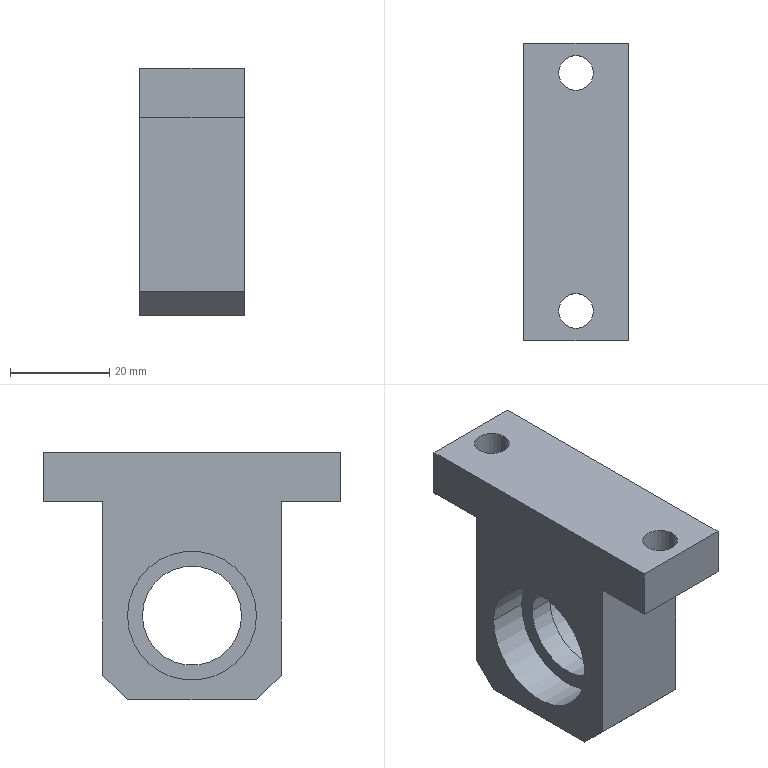Component | SolidWorks | VerticalFrontSeat-2-1 | 1 solid | 24 faces | box 21 x 60 x 50 mm | volume 31480 mm3 | plane 14 | cylinder 10 | commonest cylinder face diameters 7 x4 26 x4 20 x2
build123d program:
from build123d import *

# Parameters (mm, degrees)
SKETCH1_R           = 10
BOSS_EXTRUDE1_DEPTH = 21
SKETCH2_R           = 13
CUT_EXTRUDE1_DEPTH  = 8
CUT_EXTRUDE2_START  = -8
SKETCH3_R           = 13
CUT_EXTRUDE2_DEPTH  = 8
CHAMFER1_SIZE       = 5
SKETCH4_R           = 3.5
CUT_EXTRUDE3_DEPTH  = 12


with BuildPart() as part:
    # Sketch1 → Boss-Extrude1 (new body)
    with BuildSketch(Plane.XY):
        Polygon((12, 50), (12, 10), (0, 10), (0, 0), (60, 0), (60, 10), (48, 10), (48, 50), align=None)
        with Locations(Location((30, 33, 0), (0, 0, 180))):
            Circle(SKETCH1_R, mode=Mode.SUBTRACT)
    extrude(amount=BOSS_EXTRUDE1_DEPTH)

    # Sketch2 → Cut-Extrude1 (cut)
    with BuildSketch(Plane.XY.offset(21)):
        with Locations((30, 33)):
            Circle(SKETCH2_R)
    extrude(amount=-CUT_EXTRUDE1_DEPTH, mode=Mode.SUBTRACT)

    # Sketch3 → Cut-Extrude2 (cut)
    with BuildSketch(Plane(origin=(0, 0, 0), x_dir=(-1, 0, 0), z_dir=(0, 0, -1)).offset(CUT_EXTRUDE2_START)):
        with Locations(Location((-30, 33, 0), (0, 0, 180))):
            Circle(SKETCH3_R)
    extrude(amount=CUT_EXTRUDE2_DEPTH, mode=Mode.SUBTRACT)

    # Chamfer1
    chamfer1_edges = [part.edges().sort_by_distance(p)[0] for p in [
        (12, 50, 10.5),
        (48, 50, 10.5),
    ]]
    chamfer(chamfer1_edges, length=CHAMFER1_SIZE)

    # Sketch4 → Cut-Extrude3 (cut)
    with BuildSketch(Plane(origin=(0, 10, 0), x_dir=(1, 0, 0), z_dir=(0, 1, 0))):
        with Locations(Location((54, -10.5, 0), (0, 0, 270))):
            Circle(SKETCH4_R)
        with Locations(Location((6, -10.5, 0), (0, 0, 270))):
            Circle(SKETCH4_R)
    extrude(amount=-CUT_EXTRUDE3_DEPTH, mode=Mode.SUBTRACT)


solid = part.part

# Placed as in the assembly
solid = solid.moved(Location((28.978, 49.945, 36.551), (-90, 90, 0)))
STEP:
#1=COLOUR_RGB('',0.7922,0.8196,0.9333);
#2=FILL_AREA_STYLE_COLOUR('',#1);
#3=FILL_AREA_STYLE('',(#2));
#4=SURFACE_STYLE_FILL_AREA(#3);
#5=SURFACE_SIDE_STYLE('',(#4));
#6=SURFACE_STYLE_USAGE(.BOTH.,#5);
#7=PRESENTATION_STYLE_ASSIGNMENT((#6));
#8=CARTESIAN_POINT('',(1.692,-0.1596,1.439));
#9=VERTEX_POINT('',#8);
#10=CARTESIAN_POINT('',(1.416,-0.1596,1.439));
#11=VERTEX_POINT('',#10);
#12=CARTESIAN_POINT('',(1.554,-0.1596,1.439));
#13=DIRECTION('',(0.,0.,-1.));
#14=DIRECTION('',(-1.,0.,0.));
#15=AXIS2_PLACEMENT_3D('',#12,#13,#14);
#16=CIRCLE('',#15,0.1378);
#17=EDGE_CURVE('',#9,#11,#16,.T.);
#18=ORIENTED_EDGE('',*,*,#17,.F.);
#19=CARTESIAN_POINT('',(1.692,-0.1596,1.045));
#20=VERTEX_POINT('',#19);
#21=CARTESIAN_POINT('',(1.692,-0.1596,1.518));
#22=DIRECTION('',(0.,0.,-1.));
#23=VECTOR('',#22,39.37);
#24=LINE('',#21,#23);
#25=EDGE_CURVE('',#9,#20,#24,.T.);
#26=ORIENTED_EDGE('',*,*,#25,.T.);
#27=CARTESIAN_POINT('',(1.416,-0.1596,1.045));
#28=VERTEX_POINT('',#27);
#29=CARTESIAN_POINT('',(1.554,-0.1596,1.045));
#30=DIRECTION('',(0.,0.,-1.));
#31=DIRECTION('',(-1.,0.,0.));
#32=AXIS2_PLACEMENT_3D('',#29,#30,#31);
#33=CIRCLE('',#32,0.1378);
#34=EDGE_CURVE('',#20,#28,#33,.T.);
#35=ORIENTED_EDGE('',*,*,#34,.T.);
#36=CARTESIAN_POINT('',(1.416,-0.1596,1.518));
#37=DIRECTION('',(0.,0.,-1.));
#38=VECTOR('',#37,39.37);
#39=LINE('',#36,#38);
#40=EDGE_CURVE('',#11,#28,#39,.T.);
#41=ORIENTED_EDGE('',*,*,#40,.F.);
#42=EDGE_LOOP('',(#18,#26,#35,#41));
#43=FACE_OUTER_BOUND('',#42,.T.);
#44=CARTESIAN_POINT('',(1.554,-0.1596,1.518));
#45=DIRECTION('',(0.,0.,-1.));
#46=DIRECTION('',(-1.,0.,0.));
#47=AXIS2_PLACEMENT_3D('',#44,#45,#46);
#48=CYLINDRICAL_SURFACE('',#47,0.1378);
#49=ADVANCED_FACE('',(#43),#48,.F.);
#50=CARTESIAN_POINT('',(1.692,1.73,1.439));
#51=VERTEX_POINT('',#50);
#52=CARTESIAN_POINT('',(1.416,1.73,1.439));
#53=VERTEX_POINT('',#52);
#54=CARTESIAN_POINT('',(1.554,1.73,1.439));
#55=DIRECTION('',(0.,0.,-1.));
#56=DIRECTION('',(-1.,0.,0.));
#57=AXIS2_PLACEMENT_3D('',#54,#55,#56);
#58=CIRCLE('',#57,0.1378);
#59=EDGE_CURVE('',#51,#53,#58,.T.);
#60=ORIENTED_EDGE('',*,*,#59,.F.);
#61=CARTESIAN_POINT('',(1.692,1.73,1.045));
#62=VERTEX_POINT('',#61);
#63=CARTESIAN_POINT('',(1.692,1.73,1.518));
#64=DIRECTION('',(0.,0.,-1.));
#65=VECTOR('',#64,39.37);
#66=LINE('',#63,#65);
#67=EDGE_CURVE('',#51,#62,#66,.T.);
#68=ORIENTED_EDGE('',*,*,#67,.T.);
#69=CARTESIAN_POINT('',(1.416,1.73,1.045));
#70=VERTEX_POINT('',#69);
#71=CARTESIAN_POINT('',(1.554,1.73,1.045));
#72=DIRECTION('',(0.,0.,-1.));
#73=DIRECTION('',(-1.,0.,0.));
#74=AXIS2_PLACEMENT_3D('',#71,#72,#73);
#75=CIRCLE('',#74,0.1378);
#76=EDGE_CURVE('',#62,#70,#75,.T.);
#77=ORIENTED_EDGE('',*,*,#76,.T.);
#78=CARTESIAN_POINT('',(1.416,1.73,1.518));
#79=DIRECTION('',(0.,0.,-1.));
#80=VECTOR('',#79,39.37);
#81=LINE('',#78,#80);
#82=EDGE_CURVE('',#53,#70,#81,.T.);
#83=ORIENTED_EDGE('',*,*,#82,.F.);
#84=EDGE_LOOP('',(#60,#68,#77,#83));
#85=FACE_OUTER_BOUND('',#84,.T.);
#86=CARTESIAN_POINT('',(1.554,1.73,1.518));
#87=DIRECTION('',(0.,0.,-1.));
#88=DIRECTION('',(-1.,0.,0.));
#89=AXIS2_PLACEMENT_3D('',#86,#87,#88);
#90=CYLINDRICAL_SURFACE('',#89,0.1378);
#91=ADVANCED_FACE('',(#85),#90,.F.);
#92=CARTESIAN_POINT('',(1.653,1.297,0.1398));
#93=VERTEX_POINT('',#92);
#94=CARTESIAN_POINT('',(1.653,0.2734,0.1398));
#95=VERTEX_POINT('',#94);
#96=CARTESIAN_POINT('',(1.653,0.7853,0.1398));
#97=DIRECTION('',(1.,-0.,0.));
#98=DIRECTION('',(0.,-1.,-0.));
#99=AXIS2_PLACEMENT_3D('',#96,#97,#98);
#100=CIRCLE('',#99,0.5118);
#101=EDGE_CURVE('',#93,#95,#100,.T.);
#102=ORIENTED_EDGE('',*,*,#101,.F.);
#103=CARTESIAN_POINT('',(1.968,1.297,0.1398));
#104=VERTEX_POINT('',#103);
#105=CARTESIAN_POINT('',(1.653,1.297,0.1398));
#106=DIRECTION('',(1.,-0.,0.));
#107=VECTOR('',#106,39.37);
#108=LINE('',#105,#107);
#109=EDGE_CURVE('',#93,#104,#108,.T.);
#110=ORIENTED_EDGE('',*,*,#109,.T.);
#111=CARTESIAN_POINT('',(1.968,0.2734,0.1398));
#112=VERTEX_POINT('',#111);
#113=CARTESIAN_POINT('',(1.968,0.7853,0.1398));
#114=DIRECTION('',(1.,-0.,0.));
#115=DIRECTION('',(0.,-1.,-0.));
#116=AXIS2_PLACEMENT_3D('',#113,#114,#115);
#117=CIRCLE('',#116,0.5118);
#118=EDGE_CURVE('',#104,#112,#117,.T.);
#119=ORIENTED_EDGE('',*,*,#118,.T.);
#120=CARTESIAN_POINT('',(1.653,0.2734,0.1398));
#121=DIRECTION('',(1.,-0.,0.));
#122=VECTOR('',#121,39.37);
#123=LINE('',#120,#122);
#124=EDGE_CURVE('',#95,#112,#123,.T.);
#125=ORIENTED_EDGE('',*,*,#124,.F.);
#126=EDGE_LOOP('',(#102,#110,#119,#125));
#127=FACE_OUTER_BOUND('',#126,.T.);
#128=CARTESIAN_POINT('',(1.653,0.7853,0.1398));
#129=DIRECTION('',(1.,-0.,0.));
#130=DIRECTION('',(0.,-1.,-0.));
#131=AXIS2_PLACEMENT_3D('',#128,#129,#130);
#132=CYLINDRICAL_SURFACE('',#131,0.5118);
#133=ADVANCED_FACE('',(#127),#132,.F.);
#134=CARTESIAN_POINT('',(1.456,0.2734,0.1398));
#135=VERTEX_POINT('',#134);
#136=CARTESIAN_POINT('',(1.456,1.297,0.1398));
#137=VERTEX_POINT('',#136);
#138=CARTESIAN_POINT('',(1.456,0.7853,0.1398));
#139=DIRECTION('',(-1.,0.,-0.));
#140=DIRECTION('',(0.,1.,0.));
#141=AXIS2_PLACEMENT_3D('',#138,#139,#140);
#142=CIRCLE('',#141,0.5118);
#143=EDGE_CURVE('',#135,#137,#142,.T.);
#144=ORIENTED_EDGE('',*,*,#143,.F.);
#145=CARTESIAN_POINT('',(1.141,0.2734,0.1398));
#146=VERTEX_POINT('',#145);
#147=CARTESIAN_POINT('',(1.456,0.2734,0.1398));
#148=DIRECTION('',(-1.,0.,-0.));
#149=VECTOR('',#148,39.37);
#150=LINE('',#147,#149);
#151=EDGE_CURVE('',#135,#146,#150,.T.);
#152=ORIENTED_EDGE('',*,*,#151,.T.);
#153=CARTESIAN_POINT('',(1.141,1.297,0.1398));
#154=VERTEX_POINT('',#153);
#155=CARTESIAN_POINT('',(1.141,0.7853,0.1398));
#156=DIRECTION('',(-1.,0.,-0.));
#157=DIRECTION('',(0.,1.,0.));
#158=AXIS2_PLACEMENT_3D('',#155,#156,#157);
#159=CIRCLE('',#158,0.5118);
#160=EDGE_CURVE('',#146,#154,#159,.T.);
#161=ORIENTED_EDGE('',*,*,#160,.T.);
#162=CARTESIAN_POINT('',(1.456,1.297,0.1398));
#163=DIRECTION('',(-1.,0.,-0.));
#164=VECTOR('',#163,39.37);
#165=LINE('',#162,#164);
#166=EDGE_CURVE('',#137,#154,#165,.T.);
#167=ORIENTED_EDGE('',*,*,#166,.F.);
#168=EDGE_LOOP('',(#144,#152,#161,#167));
#169=FACE_OUTER_BOUND('',#168,.T.);
#170=CARTESIAN_POINT('',(1.456,0.7853,0.1398));
#171=DIRECTION('',(-1.,0.,-0.));
#172=DIRECTION('',(0.,1.,0.));
#173=AXIS2_PLACEMENT_3D('',#170,#171,#172);
#174=CYLINDRICAL_SURFACE('',#173,0.5118);
#175=ADVANCED_FACE('',(#169),#174,.F.);
#176=CARTESIAN_POINT('',(1.456,0.3916,0.1398));
#177=VERTEX_POINT('',#176);
#178=CARTESIAN_POINT('',(1.456,1.179,0.1398));
#179=VERTEX_POINT('',#178);
#180=CARTESIAN_POINT('',(1.456,0.7853,0.1398));
#181=DIRECTION('',(-1.,0.,-0.));
#182=DIRECTION('',(0.,1.,0.));
#183=AXIS2_PLACEMENT_3D('',#180,#181,#182);
#184=CIRCLE('',#183,0.3937);
#185=EDGE_CURVE('',#177,#179,#184,.T.);
#186=ORIENTED_EDGE('',*,*,#185,.T.);
#187=CARTESIAN_POINT('',(1.653,1.179,0.1398));
#188=VERTEX_POINT('',#187);
#189=CARTESIAN_POINT('',(1.141,1.179,0.1398));
#190=DIRECTION('',(1.,-0.,0.));
#191=VECTOR('',#190,39.37);
#192=LINE('',#189,#191);
#193=EDGE_CURVE('',#179,#188,#192,.T.);
#194=ORIENTED_EDGE('',*,*,#193,.T.);
#195=CARTESIAN_POINT('',(1.653,0.3916,0.1398));
#196=VERTEX_POINT('',#195);
#197=CARTESIAN_POINT('',(1.653,0.7853,0.1398));
#198=DIRECTION('',(1.,-0.,0.));
#199=DIRECTION('',(0.,-1.,0.));
#200=AXIS2_PLACEMENT_3D('',#197,#198,#199);
#201=CIRCLE('',#200,0.3937);
#202=EDGE_CURVE('',#188,#196,#201,.T.);
#203=ORIENTED_EDGE('',*,*,#202,.T.);
#204=CARTESIAN_POINT('',(1.141,0.3916,0.1398));
#205=DIRECTION('',(1.,-0.,0.));
#206=VECTOR('',#205,39.37);
#207=LINE('',#204,#206);
#208=EDGE_CURVE('',#177,#196,#207,.T.);
#209=ORIENTED_EDGE('',*,*,#208,.F.);
#210=EDGE_LOOP('',(#186,#194,#203,#209));
#211=FACE_OUTER_BOUND('',#210,.T.);
#212=CARTESIAN_POINT('',(1.141,0.7853,0.1398));
#213=DIRECTION('',(1.,-0.,0.));
#214=DIRECTION('',(0.,-1.,0.));
#215=AXIS2_PLACEMENT_3D('',#212,#213,#214);
#216=CYLINDRICAL_SURFACE('',#215,0.3937);
#217=ADVANCED_FACE('',(#211),#216,.F.);
#218=ORIENTED_EDGE('',*,*,#193,.F.);
#219=CARTESIAN_POINT('',(1.456,0.7853,0.1398));
#220=DIRECTION('',(-1.,0.,-0.));
#221=DIRECTION('',(0.,1.,0.));
#222=AXIS2_PLACEMENT_3D('',#219,#220,#221);
#223=CIRCLE('',#222,0.3937);
#224=EDGE_CURVE('',#179,#177,#223,.T.);
#225=ORIENTED_EDGE('',*,*,#224,.T.);
#226=ORIENTED_EDGE('',*,*,#208,.T.);
#227=CARTESIAN_POINT('',(1.653,0.7853,0.1398));
#228=DIRECTION('',(1.,-0.,0.));
#229=DIRECTION('',(0.,-1.,0.));
#230=AXIS2_PLACEMENT_3D('',#227,#228,#229);
#231=CIRCLE('',#230,0.3937);
#232=EDGE_CURVE('',#196,#188,#231,.T.);
#233=ORIENTED_EDGE('',*,*,#232,.T.);
#234=EDGE_LOOP('',(#218,#225,#226,#233));
#235=FACE_OUTER_BOUND('',#234,.T.);
#236=CARTESIAN_POINT('',(1.141,0.7853,0.1398));
#237=DIRECTION('',(1.,-0.,0.));
#238=DIRECTION('',(0.,-1.,0.));
#239=AXIS2_PLACEMENT_3D('',#236,#237,#238);
#240=CYLINDRICAL_SURFACE('',#239,0.3937);
#241=ADVANCED_FACE('',(#235),#240,.F.);
#242=CARTESIAN_POINT('',(1.141,0.7853,0.1398));
#243=DIRECTION('',(-1.,0.,-0.));
#244=DIRECTION('',(0.,1.,0.));
#245=AXIS2_PLACEMENT_3D('',#242,#243,#244);
#246=CIRCLE('',#245,0.5118);
#247=EDGE_CURVE('',#154,#146,#246,.T.);
#248=ORIENTED_EDGE('',*,*,#247,.F.);
#249=ORIENTED_EDGE('',*,*,#160,.F.);
#250=EDGE_LOOP('',(#248,#249));
#251=FACE_BOUND('',#250,.T.);
#252=CARTESIAN_POINT('',(1.141,1.297,-0.5295));
#253=VERTEX_POINT('',#252);
#254=CARTESIAN_POINT('',(1.141,0.2734,-0.5295));
#255=VERTEX_POINT('',#254);
#256=CARTESIAN_POINT('',(1.141,0.07659,-0.5295));
#257=DIRECTION('',(-0.,-1.,-0.));
#258=VECTOR('',#257,39.37);
#259=LINE('',#256,#258);
#260=EDGE_CURVE('',#253,#255,#259,.T.);
#261=ORIENTED_EDGE('',*,*,#260,.T.);
#262=CARTESIAN_POINT('',(1.141,0.07659,-0.3326));
#263=VERTEX_POINT('',#262);
#264=CARTESIAN_POINT('',(1.141,-1.045,0.7894));
#265=DIRECTION('',(-0.,-0.7071,0.7071));
#266=VECTOR('',#265,39.37);
#267=LINE('',#264,#266);
#268=EDGE_CURVE('',#255,#263,#267,.T.);
#269=ORIENTED_EDGE('',*,*,#268,.T.);
#270=CARTESIAN_POINT('',(1.141,0.07659,1.045));
#271=VERTEX_POINT('',#270);
#272=CARTESIAN_POINT('',(1.141,0.07659,-0.5295));
#273=DIRECTION('',(-0.,0.,1.));
#274=VECTOR('',#273,39.37);
#275=LINE('',#272,#274);
#276=EDGE_CURVE('',#263,#271,#275,.T.);
#277=ORIENTED_EDGE('',*,*,#276,.T.);
#278=CARTESIAN_POINT('',(1.141,-0.3959,1.045));
#279=VERTEX_POINT('',#278);
#280=CARTESIAN_POINT('',(1.141,0.07659,1.045));
#281=DIRECTION('',(-0.,-1.,0.));
#282=VECTOR('',#281,39.37);
#283=LINE('',#280,#282);
#284=EDGE_CURVE('',#271,#279,#283,.T.);
#285=ORIENTED_EDGE('',*,*,#284,.T.);
#286=CARTESIAN_POINT('',(1.141,-0.3959,1.439));
#287=VERTEX_POINT('',#286);
#288=CARTESIAN_POINT('',(1.141,-0.3959,1.439));
#289=DIRECTION('',(-0.,-0.,1.));
#290=VECTOR('',#289,39.37);
#291=LINE('',#288,#290);
#292=EDGE_CURVE('',#279,#287,#291,.T.);
#293=ORIENTED_EDGE('',*,*,#292,.T.);
#294=CARTESIAN_POINT('',(1.141,1.966,1.439));
#295=VERTEX_POINT('',#294);
#296=CARTESIAN_POINT('',(1.141,-0.3959,1.439));
#297=DIRECTION('',(0.,1.,0.));
#298=VECTOR('',#297,39.37);
#299=LINE('',#296,#298);
#300=EDGE_CURVE('',#287,#295,#299,.T.);
#301=ORIENTED_EDGE('',*,*,#300,.T.);
#302=CARTESIAN_POINT('',(1.141,1.966,1.045));
#303=VERTEX_POINT('',#302);
#304=CARTESIAN_POINT('',(1.141,1.966,1.439));
#305=DIRECTION('',(0.,0.,-1.));
#306=VECTOR('',#305,39.37);
#307=LINE('',#304,#306);
#308=EDGE_CURVE('',#295,#303,#307,.T.);
#309=ORIENTED_EDGE('',*,*,#308,.T.);
#310=CARTESIAN_POINT('',(1.141,1.494,1.045));
#311=VERTEX_POINT('',#310);
#312=CARTESIAN_POINT('',(1.141,1.494,1.045));
#313=DIRECTION('',(-0.,-1.,-0.));
#314=VECTOR('',#313,39.37);
#315=LINE('',#312,#314);
#316=EDGE_CURVE('',#303,#311,#315,.T.);
#317=ORIENTED_EDGE('',*,*,#316,.T.);
#318=CARTESIAN_POINT('',(1.141,1.494,-0.3326));
#319=VERTEX_POINT('',#318);
#320=CARTESIAN_POINT('',(1.141,1.494,-0.5295));
#321=DIRECTION('',(0.,-0.,-1.));
#322=VECTOR('',#321,39.37);
#323=LINE('',#320,#322);
#324=EDGE_CURVE('',#311,#319,#323,.T.);
#325=ORIENTED_EDGE('',*,*,#324,.T.);
#326=CARTESIAN_POINT('',(1.141,1.435,-0.3917));
#327=DIRECTION('',(-0.,-0.7071,-0.7071));
#328=VECTOR('',#327,39.37);
#329=LINE('',#326,#328);
#330=EDGE_CURVE('',#319,#253,#329,.T.);
#331=ORIENTED_EDGE('',*,*,#330,.T.);
#332=EDGE_LOOP('',(#261,#269,#277,#285,#293,#301,#309,#317,#325,#331));
#333=FACE_OUTER_BOUND('',#332,.T.);
#334=CARTESIAN_POINT('',(1.141,-0.3959,1.439));
#335=DIRECTION('',(-1.,0.,-0.));
#336=DIRECTION('',(0.,1.,0.));
#337=AXIS2_PLACEMENT_3D('',#334,#335,#336);
#338=PLANE('',#337);
#339=ADVANCED_FACE('',(#251,#333),#338,.T.);
#340=CARTESIAN_POINT('',(1.968,0.7853,0.1398));
#341=DIRECTION('',(1.,-0.,0.));
#342=DIRECTION('',(0.,-1.,-0.));
#343=AXIS2_PLACEMENT_3D('',#340,#341,#342);
#344=CIRCLE('',#343,0.5118);
#345=EDGE_CURVE('',#112,#104,#344,.T.);
#346=ORIENTED_EDGE('',*,*,#345,.F.);
#347=ORIENTED_EDGE('',*,*,#118,.F.);
#348=EDGE_LOOP('',(#346,#347));
#349=FACE_BOUND('',#348,.T.);
#350=CARTESIAN_POINT('',(1.968,0.07659,-0.3326));
#351=VERTEX_POINT('',#350);
#352=CARTESIAN_POINT('',(1.968,0.07659,1.045));
#353=VERTEX_POINT('',#352);
#354=CARTESIAN_POINT('',(1.968,0.07659,-0.5295));
#355=DIRECTION('',(-0.,0.,1.));
#356=VECTOR('',#355,39.37);
#357=LINE('',#354,#356);
#358=EDGE_CURVE('',#351,#353,#357,.T.);
#359=ORIENTED_EDGE('',*,*,#358,.F.);
#360=CARTESIAN_POINT('',(1.968,0.2734,-0.5295));
#361=VERTEX_POINT('',#360);
#362=CARTESIAN_POINT('',(1.968,0.07659,-0.3326));
#363=DIRECTION('',(0.,0.7071,-0.7071));
#364=VECTOR('',#363,39.37);
#365=LINE('',#362,#364);
#366=EDGE_CURVE('',#351,#361,#365,.T.);
#367=ORIENTED_EDGE('',*,*,#366,.T.);
#368=CARTESIAN_POINT('',(1.968,1.297,-0.5295));
#369=VERTEX_POINT('',#368);
#370=CARTESIAN_POINT('',(1.968,0.07659,-0.5295));
#371=DIRECTION('',(-0.,-1.,-0.));
#372=VECTOR('',#371,39.37);
#373=LINE('',#370,#372);
#374=EDGE_CURVE('',#369,#361,#373,.T.);
#375=ORIENTED_EDGE('',*,*,#374,.F.);
#376=CARTESIAN_POINT('',(1.968,1.494,-0.3326));
#377=VERTEX_POINT('',#376);
#378=CARTESIAN_POINT('',(1.968,1.297,-0.5295));
#379=DIRECTION('',(0.,0.7071,0.7071));
#380=VECTOR('',#379,39.37);
#381=LINE('',#378,#380);
#382=EDGE_CURVE('',#369,#377,#381,.T.);
#383=ORIENTED_EDGE('',*,*,#382,.T.);
#384=CARTESIAN_POINT('',(1.968,1.494,1.045));
#385=VERTEX_POINT('',#384);
#386=CARTESIAN_POINT('',(1.968,1.494,-0.5295));
#387=DIRECTION('',(0.,-0.,-1.));
#388=VECTOR('',#387,39.37);
#389=LINE('',#386,#388);
#390=EDGE_CURVE('',#385,#377,#389,.T.);
#391=ORIENTED_EDGE('',*,*,#390,.F.);
#392=CARTESIAN_POINT('',(1.968,1.966,1.045));
#393=VERTEX_POINT('',#392);
#394=CARTESIAN_POINT('',(1.968,1.494,1.045));
#395=DIRECTION('',(-0.,-1.,-0.));
#396=VECTOR('',#395,39.37);
#397=LINE('',#394,#396);
#398=EDGE_CURVE('',#393,#385,#397,.T.);
#399=ORIENTED_EDGE('',*,*,#398,.F.);
#400=CARTESIAN_POINT('',(1.968,1.966,1.439));
#401=VERTEX_POINT('',#400);
#402=CARTESIAN_POINT('',(1.968,1.966,1.439));
#403=DIRECTION('',(0.,0.,-1.));
#404=VECTOR('',#403,39.37);
#405=LINE('',#402,#404);
#406=EDGE_CURVE('',#401,#393,#405,.T.);
#407=ORIENTED_EDGE('',*,*,#406,.F.);
#408=CARTESIAN_POINT('',(1.968,-0.3959,1.439));
#409=VERTEX_POINT('',#408);
#410=CARTESIAN_POINT('',(1.968,-0.3959,1.439));
#411=DIRECTION('',(0.,1.,0.));
#412=VECTOR('',#411,39.37);
#413=LINE('',#410,#412);
#414=EDGE_CURVE('',#409,#401,#413,.T.);
#415=ORIENTED_EDGE('',*,*,#414,.F.);
#416=CARTESIAN_POINT('',(1.968,-0.3959,1.045));
#417=VERTEX_POINT('',#416);
#418=CARTESIAN_POINT('',(1.968,-0.3959,1.439));
#419=DIRECTION('',(-0.,-0.,1.));
#420=VECTOR('',#419,39.37);
#421=LINE('',#418,#420);
#422=EDGE_CURVE('',#417,#409,#421,.T.);
#423=ORIENTED_EDGE('',*,*,#422,.F.);
#424=CARTESIAN_POINT('',(1.968,0.07659,1.045));
#425=DIRECTION('',(-0.,-1.,0.));
#426=VECTOR('',#425,39.37);
#427=LINE('',#424,#426);
#428=EDGE_CURVE('',#353,#417,#427,.T.);
#429=ORIENTED_EDGE('',*,*,#428,.F.);
#430=EDGE_LOOP('',(#359,#367,#375,#383,#391,#399,#407,#415,#423,#429));
#431=FACE_OUTER_BOUND('',#430,.T.);
#432=CARTESIAN_POINT('',(1.968,-0.3959,1.439));
#433=DIRECTION('',(-1.,0.,-0.));
#434=DIRECTION('',(0.,1.,0.));
#435=AXIS2_PLACEMENT_3D('',#432,#433,#434);
#436=PLANE('',#435);
#437=ADVANCED_FACE('',(#349,#431),#436,.F.);
#438=ORIENTED_EDGE('',*,*,#422,.T.);
#439=CARTESIAN_POINT('',(1.141,-0.3959,1.439));
#440=DIRECTION('',(1.,-0.,0.));
#441=VECTOR('',#440,39.37);
#442=LINE('',#439,#441);
#443=EDGE_CURVE('',#287,#409,#442,.T.);
#444=ORIENTED_EDGE('',*,*,#443,.F.);
#445=ORIENTED_EDGE('',*,*,#292,.F.);
#446=CARTESIAN_POINT('',(1.141,-0.3959,1.045));
#447=DIRECTION('',(1.,-0.,0.));
#448=VECTOR('',#447,39.37);
#449=LINE('',#446,#448);
#450=EDGE_CURVE('',#279,#417,#449,.T.);
#451=ORIENTED_EDGE('',*,*,#450,.T.);
#452=EDGE_LOOP('',(#438,#444,#445,#451));
#453=FACE_OUTER_BOUND('',#452,.T.);
#454=CARTESIAN_POINT('',(1.141,-0.3959,1.439));
#455=DIRECTION('',(0.,1.,0.));
#456=DIRECTION('',(1.,-0.,0.));
#457=AXIS2_PLACEMENT_3D('',#454,#455,#456);
#458=PLANE('',#457);
#459=ADVANCED_FACE('',(#453),#458,.F.);
#460=CARTESIAN_POINT('',(1.554,-0.1596,1.439));
#461=DIRECTION('',(0.,0.,-1.));
#462=DIRECTION('',(-1.,0.,0.));
#463=AXIS2_PLACEMENT_3D('',#460,#461,#462);
#464=CIRCLE('',#463,0.1378);
#465=EDGE_CURVE('',#11,#9,#464,.T.);
#466=ORIENTED_EDGE('',*,*,#465,.T.);
#467=ORIENTED_EDGE('',*,*,#17,.T.);
#468=EDGE_LOOP('',(#466,#467));
#469=FACE_BOUND('',#468,.T.);
#470=CARTESIAN_POINT('',(1.554,1.73,1.439));
#471=DIRECTION('',(0.,0.,-1.));
#472=DIRECTION('',(-1.,0.,0.));
#473=AXIS2_PLACEMENT_3D('',#470,#471,#472);
#474=CIRCLE('',#473,0.1378);
#475=EDGE_CURVE('',#53,#51,#474,.T.);
#476=ORIENTED_EDGE('',*,*,#475,.T.);
#477=ORIENTED_EDGE('',*,*,#59,.T.);
#478=EDGE_LOOP('',(#476,#477));
#479=FACE_BOUND('',#478,.T.);
#480=ORIENTED_EDGE('',*,*,#414,.T.);
#481=CARTESIAN_POINT('',(1.141,1.966,1.439));
#482=DIRECTION('',(1.,-0.,0.));
#483=VECTOR('',#482,39.37);
#484=LINE('',#481,#483);
#485=EDGE_CURVE('',#295,#401,#484,.T.);
#486=ORIENTED_EDGE('',*,*,#485,.F.);
#487=ORIENTED_EDGE('',*,*,#300,.F.);
#488=ORIENTED_EDGE('',*,*,#443,.T.);
#489=EDGE_LOOP('',(#480,#486,#487,#488));
#490=FACE_OUTER_BOUND('',#489,.T.);
#491=CARTESIAN_POINT('',(1.141,-0.3959,1.439));
#492=DIRECTION('',(0.,0.,-1.));
#493=DIRECTION('',(-1.,0.,-0.));
#494=AXIS2_PLACEMENT_3D('',#491,#492,#493);
#495=PLANE('',#494);
#496=ADVANCED_FACE('',(#469,#479,#490),#495,.F.);
#497=ORIENTED_EDGE('',*,*,#406,.T.);
#498=CARTESIAN_POINT('',(1.141,1.966,1.045));
#499=DIRECTION('',(1.,-0.,0.));
#500=VECTOR('',#499,39.37);
#501=LINE('',#498,#500);
#502=EDGE_CURVE('',#303,#393,#501,.T.);
#503=ORIENTED_EDGE('',*,*,#502,.F.);
#504=ORIENTED_EDGE('',*,*,#308,.F.);
#505=ORIENTED_EDGE('',*,*,#485,.T.);
#506=EDGE_LOOP('',(#497,#503,#504,#505));
#507=FACE_OUTER_BOUND('',#506,.T.);
#508=CARTESIAN_POINT('',(1.141,1.966,1.439));
#509=DIRECTION('',(-0.,-1.,-0.));
#510=DIRECTION('',(-1.,0.,-0.));
#511=AXIS2_PLACEMENT_3D('',#508,#509,#510);
#512=PLANE('',#511);
#513=ADVANCED_FACE('',(#507),#512,.F.);
#514=CARTESIAN_POINT('',(1.554,1.73,1.045));
#515=DIRECTION('',(0.,0.,-1.));
#516=DIRECTION('',(-1.,0.,0.));
#517=AXIS2_PLACEMENT_3D('',#514,#515,#516);
#518=CIRCLE('',#517,0.1378);
#519=EDGE_CURVE('',#70,#62,#518,.T.);
#520=ORIENTED_EDGE('',*,*,#519,.F.);
#521=ORIENTED_EDGE('',*,*,#76,.F.);
#522=EDGE_LOOP('',(#520,#521));
#523=FACE_BOUND('',#522,.T.);
#524=ORIENTED_EDGE('',*,*,#398,.T.);
#525=CARTESIAN_POINT('',(1.141,1.494,1.045));
#526=DIRECTION('',(1.,-0.,0.));
#527=VECTOR('',#526,39.37);
#528=LINE('',#525,#527);
#529=EDGE_CURVE('',#311,#385,#528,.T.);
#530=ORIENTED_EDGE('',*,*,#529,.F.);
#531=ORIENTED_EDGE('',*,*,#316,.F.);
#532=ORIENTED_EDGE('',*,*,#502,.T.);
#533=EDGE_LOOP('',(#524,#530,#531,#532));
#534=FACE_OUTER_BOUND('',#533,.T.);
#535=CARTESIAN_POINT('',(1.141,1.494,1.045));
#536=DIRECTION('',(-0.,-0.,1.));
#537=DIRECTION('',(1.,-0.,0.));
#538=AXIS2_PLACEMENT_3D('',#535,#536,#537);
#539=PLANE('',#538);
#540=ADVANCED_FACE('',(#523,#534),#539,.F.);
#541=ORIENTED_EDGE('',*,*,#390,.T.);
#542=CARTESIAN_POINT('',(1.141,1.494,-0.3326));
#543=DIRECTION('',(-1.,0.,-0.));
#544=VECTOR('',#543,39.37);
#545=LINE('',#542,#544);
#546=EDGE_CURVE('',#377,#319,#545,.T.);
#547=ORIENTED_EDGE('',*,*,#546,.T.);
#548=ORIENTED_EDGE('',*,*,#324,.F.);
#549=ORIENTED_EDGE('',*,*,#529,.T.);
#550=EDGE_LOOP('',(#541,#547,#548,#549));
#551=FACE_OUTER_BOUND('',#550,.T.);
#552=CARTESIAN_POINT('',(1.141,1.494,-0.5295));
#553=DIRECTION('',(-0.,-1.,0.));
#554=DIRECTION('',(-0.,0.,1.));
#555=AXIS2_PLACEMENT_3D('',#552,#553,#554);
#556=PLANE('',#555);
#557=ADVANCED_FACE('',(#551),#556,.F.);
#558=ORIENTED_EDGE('',*,*,#374,.T.);
#559=CARTESIAN_POINT('',(1.141,0.2734,-0.5295));
#560=DIRECTION('',(-1.,0.,-0.));
#561=VECTOR('',#560,39.37);
#562=LINE('',#559,#561);
#563=EDGE_CURVE('',#361,#255,#562,.T.);
#564=ORIENTED_EDGE('',*,*,#563,.T.);
#565=ORIENTED_EDGE('',*,*,#260,.F.);
#566=CARTESIAN_POINT('',(1.141,1.297,-0.5295));
#567=DIRECTION('',(1.,-0.,0.));
#568=VECTOR('',#567,39.37);
#569=LINE('',#566,#568);
#570=EDGE_CURVE('',#253,#369,#569,.T.);
#571=ORIENTED_EDGE('',*,*,#570,.T.);
#572=EDGE_LOOP('',(#558,#564,#565,#571));
#573=FACE_OUTER_BOUND('',#572,.T.);
#574=CARTESIAN_POINT('',(1.141,0.07659,-0.5295));
#575=DIRECTION('',(-0.,-0.,1.));
#576=DIRECTION('',(1.,-0.,0.));
#577=AXIS2_PLACEMENT_3D('',#574,#575,#576);
#578=PLANE('',#577);
#579=ADVANCED_FACE('',(#573),#578,.F.);
#580=ORIENTED_EDGE('',*,*,#276,.F.);
#581=CARTESIAN_POINT('',(1.141,0.07659,-0.3326));
#582=DIRECTION('',(1.,-0.,0.));
#583=VECTOR('',#582,39.37);
#584=LINE('',#581,#583);
#585=EDGE_CURVE('',#263,#351,#584,.T.);
#586=ORIENTED_EDGE('',*,*,#585,.T.);
#587=ORIENTED_EDGE('',*,*,#358,.T.);
#588=CARTESIAN_POINT('',(1.141,0.07659,1.045));
#589=DIRECTION('',(1.,-0.,0.));
#590=VECTOR('',#589,39.37);
#591=LINE('',#588,#590);
#592=EDGE_CURVE('',#271,#353,#591,.T.);
#593=ORIENTED_EDGE('',*,*,#592,.F.);
#594=EDGE_LOOP('',(#580,#586,#587,#593));
#595=FACE_OUTER_BOUND('',#594,.T.);
#596=CARTESIAN_POINT('',(1.141,0.07659,-0.5295));
#597=DIRECTION('',(0.,1.,-0.));
#598=DIRECTION('',(0.,-0.,-1.));
#599=AXIS2_PLACEMENT_3D('',#596,#597,#598);
#600=PLANE('',#599);
#601=ADVANCED_FACE('',(#595),#600,.F.);
#602=CARTESIAN_POINT('',(1.554,-0.1596,1.045));
#603=DIRECTION('',(0.,0.,-1.));
#604=DIRECTION('',(-1.,0.,0.));
#605=AXIS2_PLACEMENT_3D('',#602,#603,#604);
#606=CIRCLE('',#605,0.1378);
#607=EDGE_CURVE('',#28,#20,#606,.T.);
#608=ORIENTED_EDGE('',*,*,#607,.F.);
#609=ORIENTED_EDGE('',*,*,#34,.F.);
#610=EDGE_LOOP('',(#608,#609));
#611=FACE_BOUND('',#610,.T.);
#612=ORIENTED_EDGE('',*,*,#428,.T.);
#613=ORIENTED_EDGE('',*,*,#450,.F.);
#614=ORIENTED_EDGE('',*,*,#284,.F.);
#615=ORIENTED_EDGE('',*,*,#592,.T.);
#616=EDGE_LOOP('',(#612,#613,#614,#615));
#617=FACE_OUTER_BOUND('',#616,.T.);
#618=CARTESIAN_POINT('',(1.141,0.07659,1.045));
#619=DIRECTION('',(-0.,0.,1.));
#620=DIRECTION('',(0.,1.,-0.));
#621=AXIS2_PLACEMENT_3D('',#618,#619,#620);
#622=PLANE('',#621);
#623=ADVANCED_FACE('',(#611,#617),#622,.F.);
#624=ORIENTED_EDGE('',*,*,#151,.F.);
#625=CARTESIAN_POINT('',(1.456,0.7853,0.1398));
#626=DIRECTION('',(-1.,0.,-0.));
#627=DIRECTION('',(0.,1.,0.));
#628=AXIS2_PLACEMENT_3D('',#625,#626,#627);
#629=CIRCLE('',#628,0.5118);
#630=EDGE_CURVE('',#137,#135,#629,.T.);
#631=ORIENTED_EDGE('',*,*,#630,.F.);
#632=ORIENTED_EDGE('',*,*,#166,.T.);
#633=ORIENTED_EDGE('',*,*,#247,.T.);
#634=EDGE_LOOP('',(#624,#631,#632,#633));
#635=FACE_OUTER_BOUND('',#634,.T.);
#636=CARTESIAN_POINT('',(1.456,0.7853,0.1398));
#637=DIRECTION('',(-1.,0.,-0.));
#638=DIRECTION('',(0.,1.,0.));
#639=AXIS2_PLACEMENT_3D('',#636,#637,#638);
#640=CYLINDRICAL_SURFACE('',#639,0.5118);
#641=ADVANCED_FACE('',(#635),#640,.F.);
#642=ORIENTED_EDGE('',*,*,#185,.F.);
#643=ORIENTED_EDGE('',*,*,#224,.F.);
#644=EDGE_LOOP('',(#642,#643));
#645=FACE_BOUND('',#644,.T.);
#646=ORIENTED_EDGE('',*,*,#630,.T.);
#647=ORIENTED_EDGE('',*,*,#143,.T.);
#648=EDGE_LOOP('',(#646,#647));
#649=FACE_OUTER_BOUND('',#648,.T.);
#650=CARTESIAN_POINT('',(1.456,0.7853,0.1398));
#651=DIRECTION('',(-1.,0.,-0.));
#652=DIRECTION('',(0.,1.,0.));
#653=AXIS2_PLACEMENT_3D('',#650,#651,#652);
#654=PLANE('',#653);
#655=ADVANCED_FACE('',(#645,#649),#654,.T.);
#656=ORIENTED_EDGE('',*,*,#109,.F.);
#657=CARTESIAN_POINT('',(1.653,0.7853,0.1398));
#658=DIRECTION('',(1.,-0.,0.));
#659=DIRECTION('',(0.,-1.,-0.));
#660=AXIS2_PLACEMENT_3D('',#657,#658,#659);
#661=CIRCLE('',#660,0.5118);
#662=EDGE_CURVE('',#95,#93,#661,.T.);
#663=ORIENTED_EDGE('',*,*,#662,.F.);
#664=ORIENTED_EDGE('',*,*,#124,.T.);
#665=ORIENTED_EDGE('',*,*,#345,.T.);
#666=EDGE_LOOP('',(#656,#663,#664,#665));
#667=FACE_OUTER_BOUND('',#666,.T.);
#668=CARTESIAN_POINT('',(1.653,0.7853,0.1398));
#669=DIRECTION('',(1.,-0.,0.));
#670=DIRECTION('',(0.,-1.,-0.));
#671=AXIS2_PLACEMENT_3D('',#668,#669,#670);
#672=CYLINDRICAL_SURFACE('',#671,0.5118);
#673=ADVANCED_FACE('',(#667),#672,.F.);
#674=ORIENTED_EDGE('',*,*,#232,.F.);
#675=ORIENTED_EDGE('',*,*,#202,.F.);
#676=EDGE_LOOP('',(#674,#675));
#677=FACE_BOUND('',#676,.T.);
#678=ORIENTED_EDGE('',*,*,#662,.T.);
#679=ORIENTED_EDGE('',*,*,#101,.T.);
#680=EDGE_LOOP('',(#678,#679));
#681=FACE_OUTER_BOUND('',#680,.T.);
#682=CARTESIAN_POINT('',(1.653,0.7853,0.1398));
#683=DIRECTION('',(1.,-0.,0.));
#684=DIRECTION('',(-0.,-1.,-0.));
#685=AXIS2_PLACEMENT_3D('',#682,#683,#684);
#686=PLANE('',#685);
#687=ADVANCED_FACE('',(#677,#681),#686,.T.);
#688=ORIENTED_EDGE('',*,*,#268,.F.);
#689=ORIENTED_EDGE('',*,*,#563,.F.);
#690=ORIENTED_EDGE('',*,*,#366,.F.);
#691=ORIENTED_EDGE('',*,*,#585,.F.);
#692=EDGE_LOOP('',(#688,#689,#690,#691));
#693=FACE_OUTER_BOUND('',#692,.T.);
#694=CARTESIAN_POINT('',(1.141,0.07659,-0.3326));
#695=DIRECTION('',(0.,0.7071,0.7071));
#696=DIRECTION('',(1.,-0.,0.));
#697=AXIS2_PLACEMENT_3D('',#694,#695,#696);
#698=PLANE('',#697);
#699=ADVANCED_FACE('',(#693),#698,.F.);
#700=ORIENTED_EDGE('',*,*,#330,.F.);
#701=ORIENTED_EDGE('',*,*,#546,.F.);
#702=ORIENTED_EDGE('',*,*,#382,.F.);
#703=ORIENTED_EDGE('',*,*,#570,.F.);
#704=EDGE_LOOP('',(#700,#701,#702,#703));
#705=FACE_OUTER_BOUND('',#704,.T.);
#706=CARTESIAN_POINT('',(1.141,1.297,-0.5295));
#707=DIRECTION('',(-0.,-0.7071,0.7071));
#708=DIRECTION('',(1.,-0.,0.));
#709=AXIS2_PLACEMENT_3D('',#706,#707,#708);
#710=PLANE('',#709);
#711=ADVANCED_FACE('',(#705),#710,.F.);
#712=ORIENTED_EDGE('',*,*,#67,.F.);
#713=ORIENTED_EDGE('',*,*,#475,.F.);
#714=ORIENTED_EDGE('',*,*,#82,.T.);
#715=ORIENTED_EDGE('',*,*,#519,.T.);
#716=EDGE_LOOP('',(#712,#713,#714,#715));
#717=FACE_OUTER_BOUND('',#716,.T.);
#718=CARTESIAN_POINT('',(1.554,1.73,1.518));
#719=DIRECTION('',(0.,0.,-1.));
#720=DIRECTION('',(-1.,0.,0.));
#721=AXIS2_PLACEMENT_3D('',#718,#719,#720);
#722=CYLINDRICAL_SURFACE('',#721,0.1378);
#723=ADVANCED_FACE('',(#717),#722,.F.);
#724=ORIENTED_EDGE('',*,*,#25,.F.);
#725=ORIENTED_EDGE('',*,*,#465,.F.);
#726=ORIENTED_EDGE('',*,*,#40,.T.);
#727=ORIENTED_EDGE('',*,*,#607,.T.);
#728=EDGE_LOOP('',(#724,#725,#726,#727));
#729=FACE_OUTER_BOUND('',#728,.T.);
#730=CARTESIAN_POINT('',(1.554,-0.1596,1.518));
#731=DIRECTION('',(0.,0.,-1.));
#732=DIRECTION('',(-1.,0.,0.));
#733=AXIS2_PLACEMENT_3D('',#730,#731,#732);
#734=CYLINDRICAL_SURFACE('',#733,0.1378);
#735=ADVANCED_FACE('',(#729),#734,.F.);
#736=CLOSED_SHELL('',(#49,#91,#133,#175,#217,#241,#339,#437,#459,#496,#513,#540,#557,#579,#601,#623,#641,#655,#673,#687,#699,#711,#723,#735));
#737=MANIFOLD_SOLID_BREP('',#736);
#738=STYLED_ITEM('',(#7),#737);
#739=PRESENTATION_LAYER_ASSIGNMENT('','',(#738));
#740=(LENGTH_UNIT()NAMED_UNIT(*)SI_UNIT($,.METRE.));
#741=LENGTH_MEASURE_WITH_UNIT(LENGTH_MEASURE(0.0254),#740);
#742=DIMENSIONAL_EXPONENTS(1.,0.,0.,0.,0.,0.,0.);
#743=(CONVERSION_BASED_UNIT('',#741)LENGTH_UNIT()NAMED_UNIT(#742));
#744=UNCERTAINTY_MEASURE_WITH_UNIT(LENGTH_MEASURE(0.00001),#743,'','');
#745=(NAMED_UNIT(*)PLANE_ANGLE_UNIT()SI_UNIT($,.RADIAN.));
#746=(NAMED_UNIT(*)SI_UNIT($,.STERADIAN.)SOLID_ANGLE_UNIT());
#747=(GEOMETRIC_REPRESENTATION_CONTEXT(3)GLOBAL_UNCERTAINTY_ASSIGNED_CONTEXT((#744))GLOBAL_UNIT_ASSIGNED_CONTEXT((#743,#745,#746))REPRESENTATION_CONTEXT('',''));
#748=MECHANICAL_DESIGN_GEOMETRIC_PRESENTATION_REPRESENTATION('',(#738),#747);
#749=CARTESIAN_POINT('',(0.,0.,0.));
#750=DIRECTION('',(0.,0.,1.));
#751=DIRECTION('',(1.,0.,0.));
#752=AXIS2_PLACEMENT_3D('',#749,#750,#751);
#753=(LENGTH_UNIT()NAMED_UNIT(*)SI_UNIT($,.METRE.));
#754=LENGTH_MEASURE_WITH_UNIT(LENGTH_MEASURE(0.0254),#753);
#755=DIMENSIONAL_EXPONENTS(1.,0.,0.,0.,0.,0.,0.);
#756=(CONVERSION_BASED_UNIT('',#754)LENGTH_UNIT()NAMED_UNIT(#755));
#757=UNCERTAINTY_MEASURE_WITH_UNIT(LENGTH_MEASURE(0.00001),#756,'','');
#758=(NAMED_UNIT(*)PLANE_ANGLE_UNIT()SI_UNIT($,.RADIAN.));
#759=(NAMED_UNIT(*)SI_UNIT($,.STERADIAN.)SOLID_ANGLE_UNIT());
#760=(GEOMETRIC_REPRESENTATION_CONTEXT(3)GLOBAL_UNCERTAINTY_ASSIGNED_CONTEXT((#757))GLOBAL_UNIT_ASSIGNED_CONTEXT((#756,#758,#759))REPRESENTATION_CONTEXT('',''));
#761=ADVANCED_BREP_SHAPE_REPRESENTATION('',(#737,#752),#760);